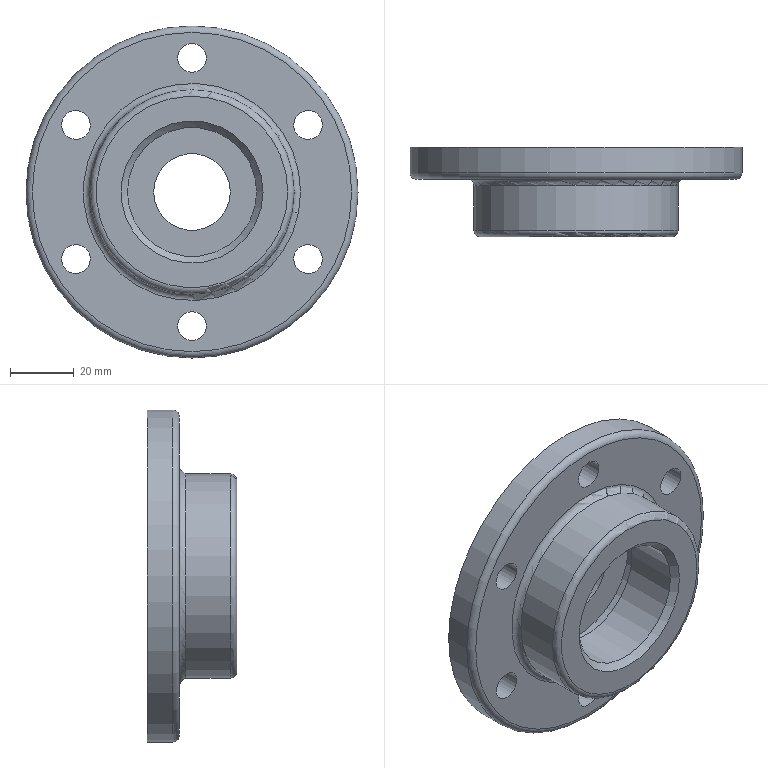Component | NX | END_CAP | 1 solid | 20 faces | volume 106215 mm3 | cylinder 11 | plane 5 | torus 3 | cone 1 | commonest cylinder face diameters 9 x6 104 x1 64 x1 40.5 x1 44 x1 24 x1